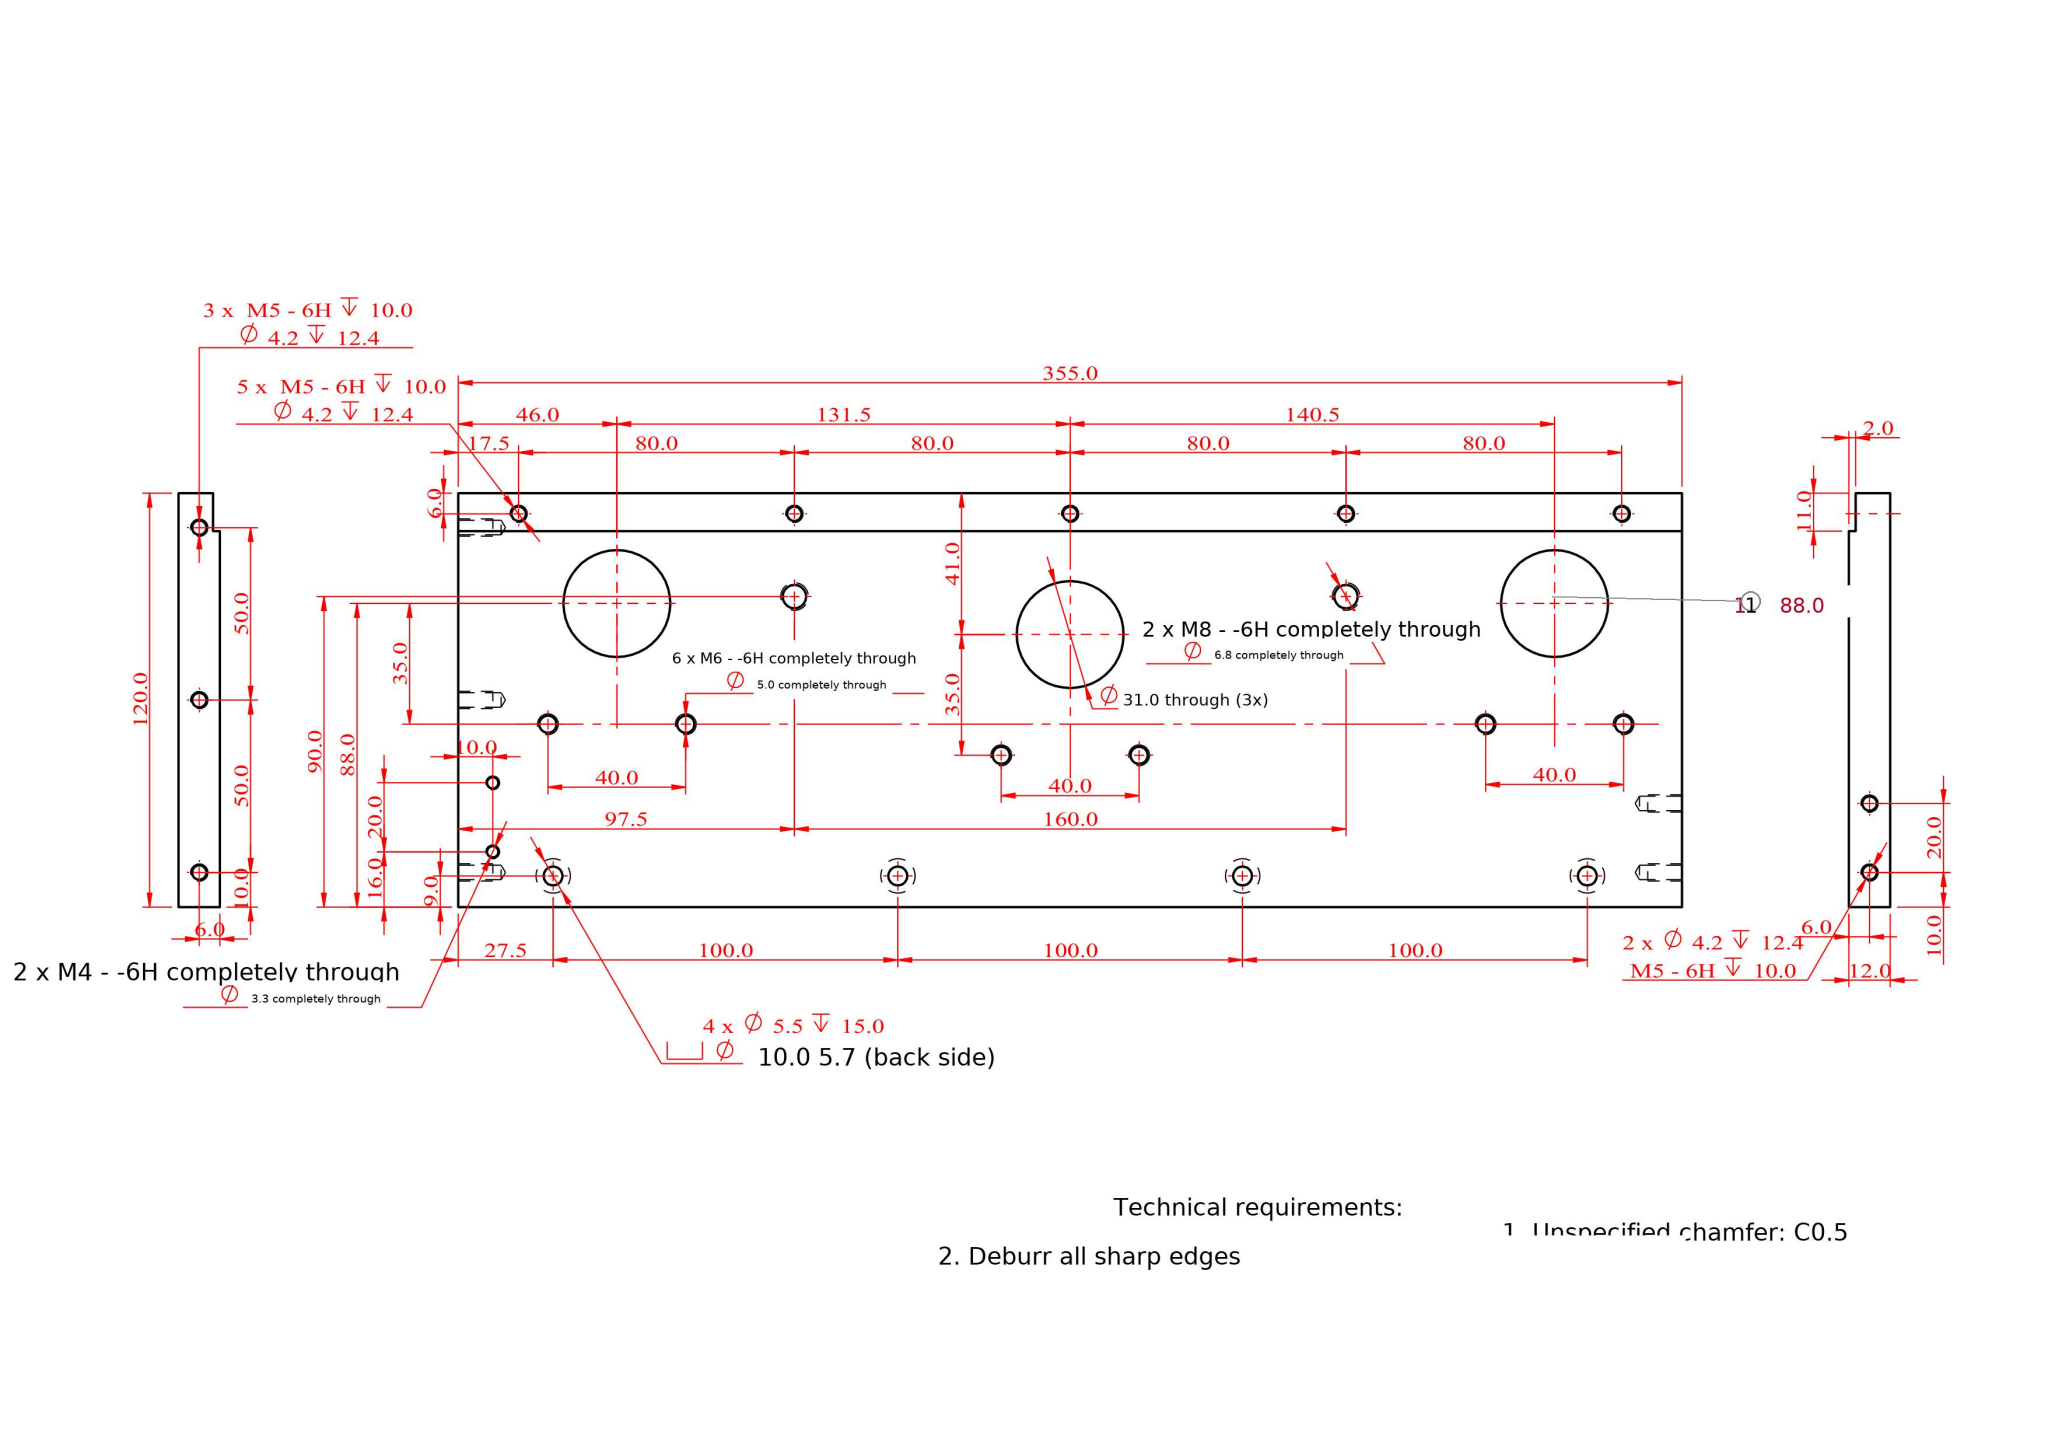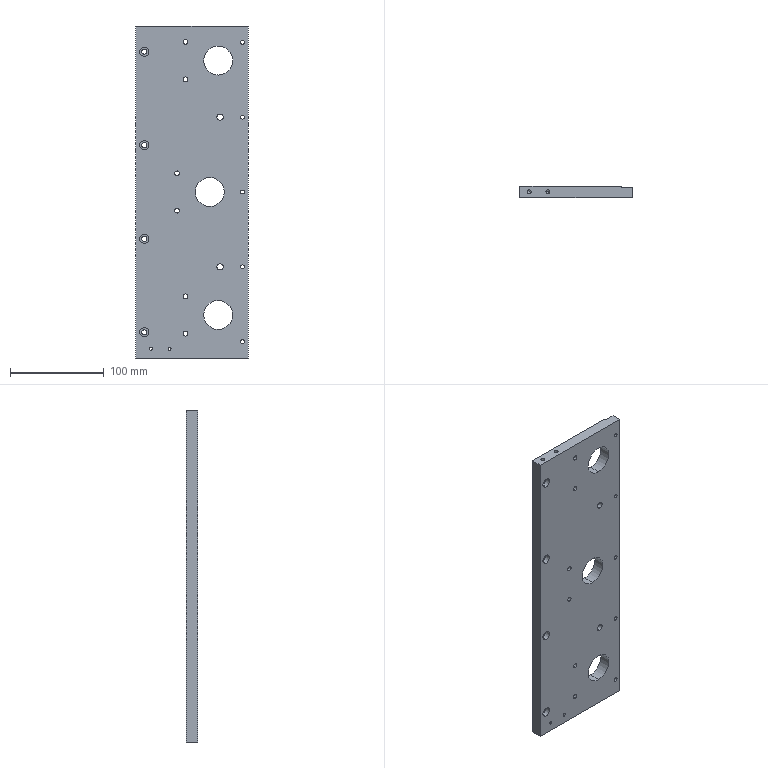Part | SolidWorks | mm | 1 solid | 84 faces | box 120 x 12 x 355 mm | volume 469758 mm3 | cylinder 62 | plane 12 | cone 10 | commonest cylinder face diameters 4.2 x20 5 x12 10 x8 5.5 x8 31 x6 3.3 x4 6.8 x4
build123d program:
from build123d import *

# Parameters (mm, degrees)
SKETCH2_W                                            = 120
SKETCH2_H                                            = 355
BOSS_EXTRUDE1_DEPTH                                  = 6
HOLE_SIZE_ACCORDING_TO_TYPE_0_OF_HEX_SOC_D           = 5.5
HOLE_SIZE_ACCORDING_TO_TYPE_0_OF_HEX_SOC_DEPTH       = 15
HOLE_SIZE_ACCORDING_TO_TYPE_0_OF_HEX_SOC_CBORE_D     = 10
HOLE_SIZE_ACCORDING_TO_TYPE_0_OF_HEX_SOC_CBORE_DEPTH = 5.7
HOLE_SIZE_ACCORDING_TO_TYPE_0_OF_HEX_SOC_TIP         = 1.652
SKETCH5_W                                            = 11
SKETCH5_H                                            = 355
CUT_EXTRUDE1_DEPTH                                   = 2
M5_TAPPED_HOLE1_D                                    = 4.2
M5_TAPPED_HOLE1_DEPTH                                = 12.4
M5_TAPPED_HOLE1_TIP                                  = 1.262
M8_TAPPED_HOLE1_D                                    = 6.8
M5_TAPPED_HOLE3_D                                    = 4.2
M5_TAPPED_HOLE3_DEPTH                                = 12.4
M5_TAPPED_HOLE3_TIP                                  = 1.262
M4_TAPPED_HOLE1_D                                    = 3.3
SKETCH25_R                                           = 15.5
CUT_EXTRUDE3_DEPTH                                   = 188.75
M5_TAPPED_HOLE5_D                                    = 4.2
M5_TAPPED_HOLE5_DEPTH                                = 12.4
M5_TAPPED_HOLE5_TIP                                  = 1.262
M6_TAPPED_HOLE1_D                                    = 5


with BuildPart() as part:
    # Sketch2 → Boss-Extrude1 (new, symmetric)
    with BuildSketch(Plane(origin=(0, 0, 0), x_dir=(1, 0, 0), z_dir=(0, 1, 0))):
        Rectangle(SKETCH2_W, SKETCH2_H)
    extrude(amount=BOSS_EXTRUDE1_DEPTH, both=True)

    # Hole Size_According to_Type 0 of Hex Soc
    with Locations(Plane(origin=(0, -6, 0), x_dir=(-1, 0, 0), z_dir=(0, -1, 0))):
        with Locations((51, -150), (51, -50), (51, 50), (51, 150)):
            CounterBoreHole(HOLE_SIZE_ACCORDING_TO_TYPE_0_OF_HEX_SOC_D / 2, HOLE_SIZE_ACCORDING_TO_TYPE_0_OF_HEX_SOC_CBORE_D / 2, HOLE_SIZE_ACCORDING_TO_TYPE_0_OF_HEX_SOC_CBORE_DEPTH, depth=HOLE_SIZE_ACCORDING_TO_TYPE_0_OF_HEX_SOC_DEPTH)
            with Locations((0, 0, -(HOLE_SIZE_ACCORDING_TO_TYPE_0_OF_HEX_SOC_DEPTH + HOLE_SIZE_ACCORDING_TO_TYPE_0_OF_HEX_SOC_TIP / 2))):  # 118° drill point
                Cone(0, HOLE_SIZE_ACCORDING_TO_TYPE_0_OF_HEX_SOC_D / 2, HOLE_SIZE_ACCORDING_TO_TYPE_0_OF_HEX_SOC_TIP, mode=Mode.SUBTRACT)

    # Sketch5 → Cut-Extrude1 (cut)
    with BuildSketch(Plane(origin=(0, 6, 0), x_dir=(1, 0, 0), z_dir=(0, 1, 0))):
        with Locations((54.5, 0)):
            Rectangle(SKETCH5_W, SKETCH5_H)
    extrude(amount=-CUT_EXTRUDE1_DEPTH, mode=Mode.SUBTRACT)

    # M5 Tapped Hole1
    with Locations(Plane(origin=(0, 0, -177.5), x_dir=(1, 0, 0), z_dir=(0, 0, -1))):
        with Locations((-50, 0), (0, 0), (50, 0)):
            Hole(M5_TAPPED_HOLE1_D / 2, depth=M5_TAPPED_HOLE1_DEPTH)
            with Locations((0, 0, -(M5_TAPPED_HOLE1_DEPTH + M5_TAPPED_HOLE1_TIP / 2))):  # 118° drill point
                Cone(0, M5_TAPPED_HOLE1_D / 2, M5_TAPPED_HOLE1_TIP, mode=Mode.SUBTRACT)

    # M8 Tapped Hole1 (through all)
    with Locations(Plane(origin=(0, -6, 0), x_dir=(-1, 0, 0), z_dir=(0, -1, 0))):
        with Locations((-30, 80), (-30, -80)):
            Hole(M8_TAPPED_HOLE1_D / 2)

    # M5 Tapped Hole3
    with Locations(Plane(origin=(0, 4, 0), x_dir=(1, 0, 0), z_dir=(0, 1, 0))):
        with Locations((54, -160), (54, -80), (54, 80), (54, 160), (54, 0)):
            Hole(M5_TAPPED_HOLE3_D / 2, depth=M5_TAPPED_HOLE3_DEPTH)
            with Locations((0, 0, -(M5_TAPPED_HOLE3_DEPTH + M5_TAPPED_HOLE3_TIP / 2))):  # 118° drill point
                Cone(0, M5_TAPPED_HOLE3_D / 2, M5_TAPPED_HOLE3_TIP, mode=Mode.SUBTRACT)

    # M4 Tapped Hole1 (through all)
    with Locations(Plane(origin=(0, -6, 0), x_dir=(-1, 0, 0), z_dir=(0, -1, 0))):
        with Locations((44, 167.5), (24, 167.5)):
            Hole(M4_TAPPED_HOLE1_D / 2)

    # Sketch25 → Cut-Extrude3 (cut, through all)
    with BuildSketch(Plane.XZ.offset(6)):
        with Locations(Location((28, -131.5, 0), (0, 0, 270))):
            Circle(SKETCH25_R)
        with Locations(Location((28, 140.5, 0), (0, 0, 270))):
            Circle(SKETCH25_R)
        with Locations(Location((19, 0, 0), (0, 0, 270))):
            Circle(SKETCH25_R)
    extrude(amount=-CUT_EXTRUDE3_DEPTH, mode=Mode.SUBTRACT)

    # M5 Tapped Hole5
    with Locations(Plane.XY.offset(177.5)):
        with Locations((-50, 0), (-30, 0)):
            Hole(M5_TAPPED_HOLE5_D / 2, depth=M5_TAPPED_HOLE5_DEPTH)
            with Locations((0, 0, -(M5_TAPPED_HOLE5_DEPTH + M5_TAPPED_HOLE5_TIP / 2))):  # 118° drill point
                Cone(0, M5_TAPPED_HOLE5_D / 2, M5_TAPPED_HOLE5_TIP, mode=Mode.SUBTRACT)

    # M6 Tapped Hole1 (through all)
    with Locations(Plane(origin=(0, -6, 0), x_dir=(-1, 0, 0), z_dir=(0, -1, 0))):
        with Locations((7, 151.5), (7, 111.5), (7, -120.5), (7, -160.5), (16, -20), (16, 20)):
            Hole(M6_TAPPED_HOLE1_D / 2)


solid = part.part